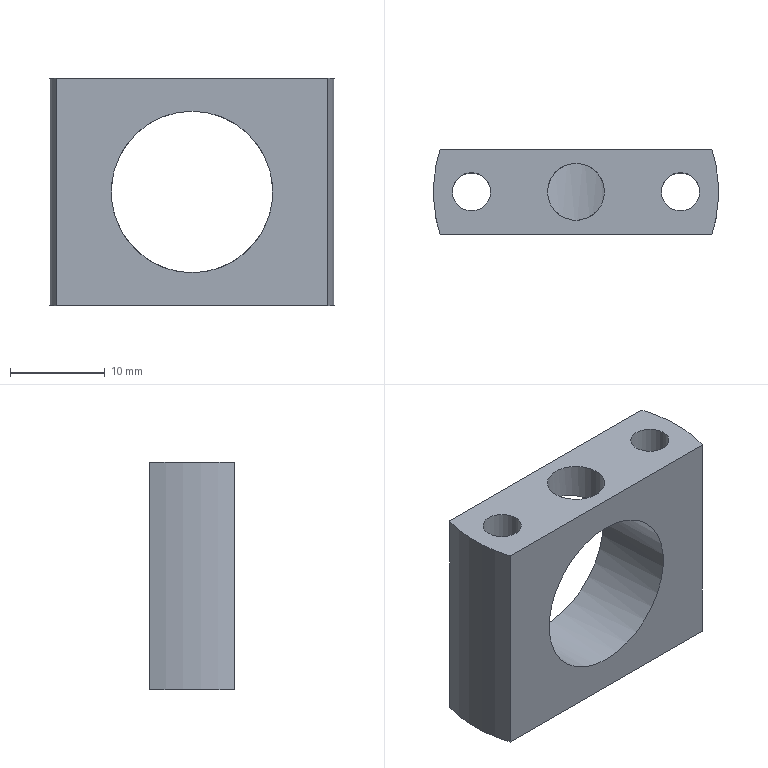Component | NX | PEDESTAL_2 | 1 solid | 10 faces | volume 3625 mm3 | cylinder 6 | plane 4 | commonest cylinder face diameters 30 x2 4.024 x2 17 x1 6 x1